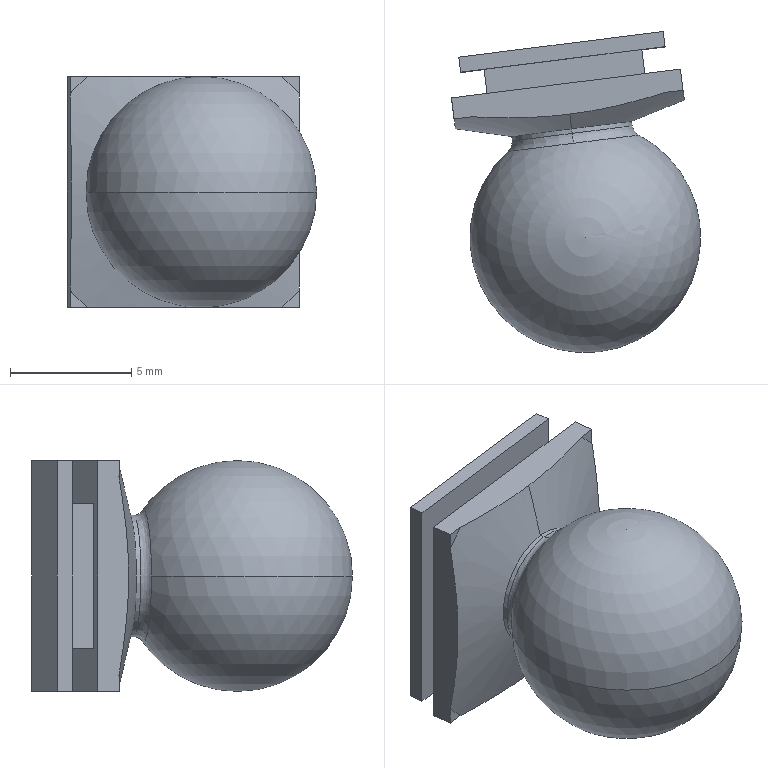Component | SolidWorks | BallJointRod-1 | 1 solid | 27 faces | box 10.26 x 13.22 x 9.5 mm | volume 678 mm3 | plane 19 | cone 2 | torus 2 | sphere 2 | cylinder 2 | commonest cylinder face diameters 5 x2
STEP:
#1=CARTESIAN_POINT('',(20.793,-12.64,5.146));
#2=VERTEX_POINT('',#1);
#3=CARTESIAN_POINT('',(20.793,-12.64,5.343));
#4=VERTEX_POINT('',#3);
#5=CARTESIAN_POINT('',(20.793,-12.64,5.245));
#6=DIRECTION('',(0.1249,-0.9922,0.));
#7=DIRECTION('',(0.,0.,-1.));
#8=AXIS2_PLACEMENT_3D('',#5,#6,#7);
#9=CIRCLE('',#8,0.09843);
#10=EDGE_CURVE('',#2,#4,#9,.T.);
#11=ORIENTED_EDGE('',*,*,#10,.F.);
#12=CARTESIAN_POINT('',(20.79,-12.616,5.058));
#13=VERTEX_POINT('',#12);
#14=CARTESIAN_POINT('',(20.788,-12.601,4.999));
#15=DIRECTION('',(-0.03232,0.2568,-0.9659));
#16=VECTOR('',#15,39.37);
#17=LINE('',#14,#16);
#18=EDGE_CURVE('',#2,#13,#17,.T.);
#19=ORIENTED_EDGE('',*,*,#18,.T.);
#20=CARTESIAN_POINT('',(20.945,-12.581,5.058));
#21=VERTEX_POINT('',#20);
#22=CARTESIAN_POINT('',(20.945,-12.581,5.058));
#23=CARTESIAN_POINT('',(20.92,-12.589,5.058));
#24=CARTESIAN_POINT('',(20.894,-12.596,5.058));
#25=CARTESIAN_POINT('',(20.842,-12.608,5.058));
#26=CARTESIAN_POINT('',(20.816,-12.613,5.058));
#27=CARTESIAN_POINT('',(20.79,-12.616,5.058));
#28=B_SPLINE_CURVE_WITH_KNOTS('',3,(#22,#23,#24,#25,#26,#27),.UNSPECIFIED.,.F.,.F.,(4,2,4),(0.,0.002023,0.004047),.UNSPECIFIED.);
#29=EDGE_CURVE('',#21,#13,#28,.T.);
#30=ORIENTED_EDGE('',*,*,#29,.F.);
#31=CARTESIAN_POINT('',(20.973,-12.577,5.086));
#32=VERTEX_POINT('',#31);
#33=CARTESIAN_POINT('',(20.788,-12.601,5.245));
#34=DIRECTION('',(-0.1249,0.9922,-0.));
#35=DIRECTION('',(-0.,-0.,-1.));
#36=AXIS2_PLACEMENT_3D('',#33,#34,#35);
#37=CIRCLE('',#36,0.2454);
#38=EDGE_CURVE('',#32,#21,#37,.T.);
#39=ORIENTED_EDGE('',*,*,#38,.F.);
#40=CARTESIAN_POINT('',(20.973,-12.577,5.403));
#41=VERTEX_POINT('',#40);
#42=CARTESIAN_POINT('',(20.973,-12.577,5.403));
#43=CARTESIAN_POINT('',(20.975,-12.586,5.351));
#44=CARTESIAN_POINT('',(20.975,-12.593,5.298));
#45=CARTESIAN_POINT('',(20.975,-12.593,5.219));
#46=CARTESIAN_POINT('',(20.975,-12.591,5.192));
#47=CARTESIAN_POINT('',(20.974,-12.586,5.139));
#48=CARTESIAN_POINT('',(20.974,-12.582,5.112));
#49=CARTESIAN_POINT('',(20.973,-12.577,5.086));
#50=B_SPLINE_CURVE_WITH_KNOTS('',3,(#42,#43,#44,#45,#46,#47,#48,#49),.UNSPECIFIED.,.F.,.F.,(4,2,2,4),(0.,0.004036,0.006054,0.008072),.UNSPECIFIED.);
#51=EDGE_CURVE('',#41,#32,#50,.T.);
#52=ORIENTED_EDGE('',*,*,#51,.F.);
#53=CARTESIAN_POINT('',(20.945,-12.581,5.432));
#54=VERTEX_POINT('',#53);
#55=CARTESIAN_POINT('',(20.788,-12.601,5.245));
#56=DIRECTION('',(-0.1249,0.9922,-0.));
#57=DIRECTION('',(-0.,-0.,-1.));
#58=AXIS2_PLACEMENT_3D('',#55,#56,#57);
#59=CIRCLE('',#58,0.2454);
#60=EDGE_CURVE('',#54,#41,#59,.T.);
#61=ORIENTED_EDGE('',*,*,#60,.F.);
#62=CARTESIAN_POINT('',(20.79,-12.616,5.432));
#63=VERTEX_POINT('',#62);
#64=CARTESIAN_POINT('',(20.79,-12.616,5.432));
#65=CARTESIAN_POINT('',(20.816,-12.613,5.432));
#66=CARTESIAN_POINT('',(20.842,-12.608,5.432));
#67=CARTESIAN_POINT('',(20.894,-12.596,5.432));
#68=CARTESIAN_POINT('',(20.92,-12.589,5.432));
#69=CARTESIAN_POINT('',(20.945,-12.581,5.432));
#70=B_SPLINE_CURVE_WITH_KNOTS('',3,(#64,#65,#66,#67,#68,#69),.UNSPECIFIED.,.F.,.F.,(4,2,4),(0.004047,0.006059,0.008072),.UNSPECIFIED.);
#71=EDGE_CURVE('',#63,#54,#70,.T.);
#72=ORIENTED_EDGE('',*,*,#71,.F.);
#73=CARTESIAN_POINT('',(20.788,-12.601,5.49));
#74=DIRECTION('',(-0.03232,0.2568,0.9659));
#75=VECTOR('',#74,39.37);
#76=LINE('',#73,#75);
#77=EDGE_CURVE('',#4,#63,#76,.T.);
#78=ORIENTED_EDGE('',*,*,#77,.F.);
#79=EDGE_LOOP('',(#11,#19,#30,#39,#52,#61,#72,#78));
#80=FACE_OUTER_BOUND('',#79,.T.);
#81=CARTESIAN_POINT('',(20.788,-12.601,5.245));
#82=DIRECTION('',(-0.1249,0.9922,-0.));
#83=DIRECTION('',(0.,0.,1.));
#84=AXIS2_PLACEMENT_3D('',#81,#82,#83);
#85=CONICAL_SURFACE('',#84,0.2454,1.309);
#86=ADVANCED_FACE('',(#80),#85,.T.);
#87=CARTESIAN_POINT('',(20.796,-12.663,5.351));
#88=VERTEX_POINT('',#87);
#89=CARTESIAN_POINT('',(20.69,-12.677,5.245));
#90=VERTEX_POINT('',#89);
#91=CARTESIAN_POINT('',(20.796,-12.663,5.245));
#92=DIRECTION('',(0.1249,-0.9922,0.));
#93=DIRECTION('',(0.,0.,-1.));
#94=AXIS2_PLACEMENT_3D('',#91,#92,#93);
#95=CIRCLE('',#94,0.1069);
#96=EDGE_CURVE('',#88,#90,#95,.T.);
#97=ORIENTED_EDGE('',*,*,#96,.F.);
#98=CARTESIAN_POINT('',(20.794,-12.647,5.343));
#99=VERTEX_POINT('',#98);
#100=CARTESIAN_POINT('',(20.794,-12.647,5.363));
#101=DIRECTION('',(0.9922,0.1249,0.));
#102=DIRECTION('',(-0.1249,0.9922,0.));
#103=AXIS2_PLACEMENT_3D('',#100,#101,#102);
#104=CIRCLE('',#103,0.01969);
#105=EDGE_CURVE('',#88,#99,#104,.T.);
#106=ORIENTED_EDGE('',*,*,#105,.T.);
#107=CARTESIAN_POINT('',(20.794,-12.647,5.146));
#108=VERTEX_POINT('',#107);
#109=CARTESIAN_POINT('',(20.794,-12.647,5.245));
#110=DIRECTION('',(-0.1249,0.9922,-0.));
#111=DIRECTION('',(0.,0.,-1.));
#112=AXIS2_PLACEMENT_3D('',#109,#110,#111);
#113=CIRCLE('',#112,0.09843);
#114=EDGE_CURVE('',#108,#99,#113,.T.);
#115=ORIENTED_EDGE('',*,*,#114,.F.);
#116=CARTESIAN_POINT('',(20.796,-12.663,5.138));
#117=VERTEX_POINT('',#116);
#118=CARTESIAN_POINT('',(20.794,-12.647,5.126));
#119=DIRECTION('',(-0.9922,-0.1249,-0.));
#120=DIRECTION('',(0.1249,-0.9922,0.));
#121=AXIS2_PLACEMENT_3D('',#118,#119,#120);
#122=CIRCLE('',#121,0.01969);
#123=EDGE_CURVE('',#117,#108,#122,.T.);
#124=ORIENTED_EDGE('',*,*,#123,.F.);
#125=CARTESIAN_POINT('',(20.796,-12.663,5.245));
#126=DIRECTION('',(0.1249,-0.9922,0.));
#127=DIRECTION('',(0.,0.,-1.));
#128=AXIS2_PLACEMENT_3D('',#125,#126,#127);
#129=CIRCLE('',#128,0.1069);
#130=EDGE_CURVE('',#90,#117,#129,.T.);
#131=ORIENTED_EDGE('',*,*,#130,.F.);
#132=EDGE_LOOP('',(#97,#106,#115,#124,#131));
#133=FACE_OUTER_BOUND('',#132,.T.);
#134=CARTESIAN_POINT('',(20.794,-12.647,5.245));
#135=DIRECTION('',(0.1249,-0.9922,0.));
#136=DIRECTION('',(0.,-0.,-1.));
#137=AXIS2_PLACEMENT_3D('',#134,#135,#136);
#138=TOROIDAL_SURFACE('',#137,0.1181,0.01969);
#139=ADVANCED_FACE('',(#133),#138,.F.);
#140=CARTESIAN_POINT('',(20.838,-13.001,5.245));
#141=VERTEX_POINT('',#140);
#142=CARTESIAN_POINT('',(20.902,-12.65,5.245));
#143=VERTEX_POINT('',#142);
#144=CARTESIAN_POINT('',(20.815,-12.815,5.245));
#145=DIRECTION('',(-0.,0.,1.));
#146=DIRECTION('',(1.,0.,0.));
#147=AXIS2_PLACEMENT_3D('',#144,#145,#146);
#148=CIRCLE('',#147,0.187);
#149=EDGE_CURVE('',#141,#143,#148,.T.);
#150=ORIENTED_EDGE('',*,*,#149,.F.);
#151=CARTESIAN_POINT('',(20.815,-12.815,5.245));
#152=DIRECTION('',(0.,-0.,-1.));
#153=DIRECTION('',(-1.,0.,0.));
#154=AXIS2_PLACEMENT_3D('',#151,#152,#153);
#155=CIRCLE('',#154,0.187);
#156=EDGE_CURVE('',#141,#90,#155,.T.);
#157=ORIENTED_EDGE('',*,*,#156,.T.);
#158=ORIENTED_EDGE('',*,*,#130,.T.);
#159=CARTESIAN_POINT('',(20.796,-12.663,5.245));
#160=DIRECTION('',(0.1249,-0.9922,0.));
#161=DIRECTION('',(0.,0.,-1.));
#162=AXIS2_PLACEMENT_3D('',#159,#160,#161);
#163=CIRCLE('',#162,0.1069);
#164=EDGE_CURVE('',#117,#143,#163,.T.);
#165=ORIENTED_EDGE('',*,*,#164,.T.);
#166=EDGE_LOOP('',(#150,#157,#158,#165));
#167=FACE_OUTER_BOUND('',#166,.T.);
#168=CARTESIAN_POINT('',(20.815,-12.815,5.245));
#169=DIRECTION('',(0.,-0.,-1.));
#170=DIRECTION('',(0.9922,0.1249,0.));
#171=AXIS2_PLACEMENT_3D('',#168,#169,#170);
#172=SPHERICAL_SURFACE('',#171,0.187);
#173=ADVANCED_FACE('',(#167),#172,.T.);
#174=ORIENTED_EDGE('',*,*,#10,.T.);
#175=CARTESIAN_POINT('',(20.788,-12.601,5.343));
#176=DIRECTION('',(0.1249,-0.9922,0.));
#177=VECTOR('',#176,39.37);
#178=LINE('',#175,#177);
#179=EDGE_CURVE('',#4,#99,#178,.T.);
#180=ORIENTED_EDGE('',*,*,#179,.T.);
#181=CARTESIAN_POINT('',(20.794,-12.647,5.245));
#182=DIRECTION('',(-0.1249,0.9922,-0.));
#183=DIRECTION('',(0.,0.,-1.));
#184=AXIS2_PLACEMENT_3D('',#181,#182,#183);
#185=CIRCLE('',#184,0.09843);
#186=EDGE_CURVE('',#99,#108,#185,.T.);
#187=ORIENTED_EDGE('',*,*,#186,.T.);
#188=CARTESIAN_POINT('',(20.788,-12.601,5.146));
#189=DIRECTION('',(0.1249,-0.9922,0.));
#190=VECTOR('',#189,39.37);
#191=LINE('',#188,#190);
#192=EDGE_CURVE('',#2,#108,#191,.T.);
#193=ORIENTED_EDGE('',*,*,#192,.F.);
#194=EDGE_LOOP('',(#174,#180,#187,#193));
#195=FACE_OUTER_BOUND('',#194,.T.);
#196=CARTESIAN_POINT('',(20.788,-12.601,5.245));
#197=DIRECTION('',(0.1249,-0.9922,0.));
#198=DIRECTION('',(0.,0.,-1.));
#199=AXIS2_PLACEMENT_3D('',#196,#197,#198);
#200=CYLINDRICAL_SURFACE('',#199,0.09843);
#201=ADVANCED_FACE('',(#195),#200,.T.);
#202=CARTESIAN_POINT('',(20.944,-12.507,5.058));
#203=VERTEX_POINT('',#202);
#204=CARTESIAN_POINT('',(20.613,-12.548,5.058));
#205=VERTEX_POINT('',#204);
#206=CARTESIAN_POINT('',(20.906,-12.511,5.058));
#207=DIRECTION('',(-0.9922,-0.1249,-0.));
#208=VECTOR('',#207,39.37);
#209=LINE('',#206,#208);
#210=EDGE_CURVE('',#203,#205,#209,.T.);
#211=ORIENTED_EDGE('',*,*,#210,.T.);
#212=CARTESIAN_POINT('',(20.61,-12.524,5.058));
#213=VERTEX_POINT('',#212);
#214=CARTESIAN_POINT('',(20.613,-12.548,5.058));
#215=DIRECTION('',(-0.1249,0.9922,-0.));
#216=VECTOR('',#215,39.37);
#217=LINE('',#214,#216);
#218=EDGE_CURVE('',#205,#213,#217,.T.);
#219=ORIENTED_EDGE('',*,*,#218,.T.);
#220=CARTESIAN_POINT('',(20.941,-12.482,5.058));
#221=VERTEX_POINT('',#220);
#222=CARTESIAN_POINT('',(20.59,-12.526,5.058));
#223=DIRECTION('',(-0.9922,-0.1249,-0.));
#224=VECTOR('',#223,39.37);
#225=LINE('',#222,#224);
#226=EDGE_CURVE('',#221,#213,#225,.T.);
#227=ORIENTED_EDGE('',*,*,#226,.F.);
#228=CARTESIAN_POINT('',(20.944,-12.507,5.058));
#229=DIRECTION('',(0.1249,-0.9922,0.));
#230=VECTOR('',#229,39.37);
#231=LINE('',#228,#230);
#232=EDGE_CURVE('',#221,#203,#231,.T.);
#233=ORIENTED_EDGE('',*,*,#232,.T.);
#234=EDGE_LOOP('',(#211,#219,#227,#233));
#235=FACE_OUTER_BOUND('',#234,.T.);
#236=CARTESIAN_POINT('',(20.59,-12.526,5.058));
#237=DIRECTION('',(-0.,0.,1.));
#238=DIRECTION('',(0.9922,0.1249,0.));
#239=AXIS2_PLACEMENT_3D('',#236,#237,#238);
#240=PLANE('',#239);
#241=ADVANCED_FACE('',(#235),#240,.F.);
#242=CARTESIAN_POINT('',(20.944,-12.507,5.432));
#243=VERTEX_POINT('',#242);
#244=CARTESIAN_POINT('',(20.613,-12.548,5.432));
#245=VERTEX_POINT('',#244);
#246=CARTESIAN_POINT('',(20.651,-12.543,5.432));
#247=DIRECTION('',(-0.9922,-0.1249,-0.));
#248=VECTOR('',#247,39.37);
#249=LINE('',#246,#248);
#250=EDGE_CURVE('',#243,#245,#249,.T.);
#251=ORIENTED_EDGE('',*,*,#250,.F.);
#252=CARTESIAN_POINT('',(20.941,-12.482,5.432));
#253=VERTEX_POINT('',#252);
#254=CARTESIAN_POINT('',(20.944,-12.507,5.432));
#255=DIRECTION('',(0.1249,-0.9922,0.));
#256=VECTOR('',#255,39.37);
#257=LINE('',#254,#256);
#258=EDGE_CURVE('',#253,#243,#257,.T.);
#259=ORIENTED_EDGE('',*,*,#258,.F.);
#260=CARTESIAN_POINT('',(20.61,-12.524,5.432));
#261=VERTEX_POINT('',#260);
#262=CARTESIAN_POINT('',(20.59,-12.526,5.432));
#263=DIRECTION('',(0.9922,0.1249,0.));
#264=VECTOR('',#263,39.37);
#265=LINE('',#262,#264);
#266=EDGE_CURVE('',#261,#253,#265,.T.);
#267=ORIENTED_EDGE('',*,*,#266,.F.);
#268=CARTESIAN_POINT('',(20.613,-12.548,5.432));
#269=DIRECTION('',(-0.1249,0.9922,-0.));
#270=VECTOR('',#269,39.37);
#271=LINE('',#268,#270);
#272=EDGE_CURVE('',#245,#261,#271,.T.);
#273=ORIENTED_EDGE('',*,*,#272,.F.);
#274=EDGE_LOOP('',(#251,#259,#267,#273));
#275=FACE_OUTER_BOUND('',#274,.T.);
#276=CARTESIAN_POINT('',(20.59,-12.526,5.432));
#277=DIRECTION('',(0.,-0.,-1.));
#278=DIRECTION('',(-0.9922,-0.1249,-0.));
#279=AXIS2_PLACEMENT_3D('',#276,#277,#278);
#280=PLANE('',#279);
#281=ADVANCED_FACE('',(#275),#280,.F.);
#282=CARTESIAN_POINT('',(20.973,-12.577,5.058));
#283=VERTEX_POINT('',#282);
#284=CARTESIAN_POINT('',(20.973,-12.577,5.432));
#285=DIRECTION('',(0.,-0.,-1.));
#286=VECTOR('',#285,39.37);
#287=LINE('',#284,#286);
#288=EDGE_CURVE('',#32,#283,#287,.T.);
#289=ORIENTED_EDGE('',*,*,#288,.F.);
#290=ORIENTED_EDGE('',*,*,#38,.T.);
#291=CARTESIAN_POINT('',(20.602,-12.624,5.058));
#292=DIRECTION('',(-0.9922,-0.1249,-0.));
#293=VECTOR('',#292,39.37);
#294=LINE('',#291,#293);
#295=EDGE_CURVE('',#283,#21,#294,.T.);
#296=ORIENTED_EDGE('',*,*,#295,.F.);
#297=EDGE_LOOP('',(#289,#290,#296));
#298=FACE_OUTER_BOUND('',#297,.T.);
#299=CARTESIAN_POINT('',(20.788,-12.601,5.245));
#300=DIRECTION('',(0.1249,-0.9922,0.));
#301=DIRECTION('',(0.,-0.,-1.));
#302=AXIS2_PLACEMENT_3D('',#299,#300,#301);
#303=PLANE('',#302);
#304=ADVANCED_FACE('',(#298),#303,.T.);
#305=CARTESIAN_POINT('',(20.63,-12.62,5.058));
#306=VERTEX_POINT('',#305);
#307=CARTESIAN_POINT('',(20.602,-12.624,5.058));
#308=VERTEX_POINT('',#307);
#309=CARTESIAN_POINT('',(20.602,-12.624,5.058));
#310=DIRECTION('',(-0.9922,-0.1249,-0.));
#311=VECTOR('',#310,39.37);
#312=LINE('',#309,#311);
#313=EDGE_CURVE('',#306,#308,#312,.T.);
#314=ORIENTED_EDGE('',*,*,#313,.F.);
#315=CARTESIAN_POINT('',(20.602,-12.624,5.086));
#316=VERTEX_POINT('',#315);
#317=CARTESIAN_POINT('',(20.788,-12.601,5.245));
#318=DIRECTION('',(-0.1249,0.9922,-0.));
#319=DIRECTION('',(0.,0.,-1.));
#320=AXIS2_PLACEMENT_3D('',#317,#318,#319);
#321=CIRCLE('',#320,0.2454);
#322=EDGE_CURVE('',#306,#316,#321,.T.);
#323=ORIENTED_EDGE('',*,*,#322,.T.);
#324=CARTESIAN_POINT('',(20.602,-12.624,5.432));
#325=DIRECTION('',(-0.,0.,1.));
#326=VECTOR('',#325,39.37);
#327=LINE('',#324,#326);
#328=EDGE_CURVE('',#308,#316,#327,.T.);
#329=ORIENTED_EDGE('',*,*,#328,.F.);
#330=EDGE_LOOP('',(#314,#323,#329));
#331=FACE_OUTER_BOUND('',#330,.T.);
#332=CARTESIAN_POINT('',(20.788,-12.601,5.245));
#333=DIRECTION('',(0.1249,-0.9922,0.));
#334=DIRECTION('',(0.,-0.,-1.));
#335=AXIS2_PLACEMENT_3D('',#332,#333,#334);
#336=PLANE('',#335);
#337=ADVANCED_FACE('',(#331),#336,.T.);
#338=CARTESIAN_POINT('',(20.602,-12.624,5.403));
#339=VERTEX_POINT('',#338);
#340=CARTESIAN_POINT('',(20.602,-12.624,5.432));
#341=VERTEX_POINT('',#340);
#342=CARTESIAN_POINT('',(20.602,-12.624,5.432));
#343=DIRECTION('',(-0.,0.,1.));
#344=VECTOR('',#343,39.37);
#345=LINE('',#342,#344);
#346=EDGE_CURVE('',#339,#341,#345,.T.);
#347=ORIENTED_EDGE('',*,*,#346,.F.);
#348=CARTESIAN_POINT('',(20.63,-12.62,5.432));
#349=VERTEX_POINT('',#348);
#350=CARTESIAN_POINT('',(20.788,-12.601,5.245));
#351=DIRECTION('',(-0.1249,0.9922,-0.));
#352=DIRECTION('',(0.,0.,-1.));
#353=AXIS2_PLACEMENT_3D('',#350,#351,#352);
#354=CIRCLE('',#353,0.2454);
#355=EDGE_CURVE('',#339,#349,#354,.T.);
#356=ORIENTED_EDGE('',*,*,#355,.T.);
#357=CARTESIAN_POINT('',(20.602,-12.624,5.432));
#358=DIRECTION('',(0.9922,0.1249,0.));
#359=VECTOR('',#358,39.37);
#360=LINE('',#357,#359);
#361=EDGE_CURVE('',#341,#349,#360,.T.);
#362=ORIENTED_EDGE('',*,*,#361,.F.);
#363=EDGE_LOOP('',(#347,#356,#362));
#364=FACE_OUTER_BOUND('',#363,.T.);
#365=CARTESIAN_POINT('',(20.788,-12.601,5.245));
#366=DIRECTION('',(0.1249,-0.9922,0.));
#367=DIRECTION('',(0.,-0.,-1.));
#368=AXIS2_PLACEMENT_3D('',#365,#366,#367);
#369=PLANE('',#368);
#370=ADVANCED_FACE('',(#364),#369,.T.);
#371=ORIENTED_EDGE('',*,*,#179,.F.);
#372=CARTESIAN_POINT('',(20.793,-12.64,5.245));
#373=DIRECTION('',(0.1249,-0.9922,0.));
#374=DIRECTION('',(0.,0.,-1.));
#375=AXIS2_PLACEMENT_3D('',#372,#373,#374);
#376=CIRCLE('',#375,0.09843);
#377=EDGE_CURVE('',#4,#2,#376,.T.);
#378=ORIENTED_EDGE('',*,*,#377,.T.);
#379=ORIENTED_EDGE('',*,*,#192,.T.);
#380=ORIENTED_EDGE('',*,*,#114,.T.);
#381=EDGE_LOOP('',(#371,#378,#379,#380));
#382=FACE_OUTER_BOUND('',#381,.T.);
#383=CARTESIAN_POINT('',(20.788,-12.601,5.245));
#384=DIRECTION('',(0.1249,-0.9922,0.));
#385=DIRECTION('',(0.,0.,-1.));
#386=AXIS2_PLACEMENT_3D('',#383,#384,#385);
#387=CYLINDRICAL_SURFACE('',#386,0.09843);
#388=ADVANCED_FACE('',(#382),#387,.T.);
#389=ORIENTED_EDGE('',*,*,#156,.F.);
#390=ORIENTED_EDGE('',*,*,#149,.T.);
#391=CARTESIAN_POINT('',(20.796,-12.663,5.245));
#392=DIRECTION('',(0.1249,-0.9922,0.));
#393=DIRECTION('',(0.,0.,-1.));
#394=AXIS2_PLACEMENT_3D('',#391,#392,#393);
#395=CIRCLE('',#394,0.1069);
#396=EDGE_CURVE('',#143,#88,#395,.T.);
#397=ORIENTED_EDGE('',*,*,#396,.T.);
#398=ORIENTED_EDGE('',*,*,#96,.T.);
#399=EDGE_LOOP('',(#389,#390,#397,#398));
#400=FACE_OUTER_BOUND('',#399,.T.);
#401=CARTESIAN_POINT('',(20.815,-12.815,5.245));
#402=DIRECTION('',(0.,-0.,-1.));
#403=DIRECTION('',(0.9922,0.1249,0.));
#404=AXIS2_PLACEMENT_3D('',#401,#402,#403);
#405=SPHERICAL_SURFACE('',#404,0.187);
#406=ADVANCED_FACE('',(#400),#405,.T.);
#407=ORIENTED_EDGE('',*,*,#105,.F.);
#408=ORIENTED_EDGE('',*,*,#396,.F.);
#409=ORIENTED_EDGE('',*,*,#164,.F.);
#410=ORIENTED_EDGE('',*,*,#123,.T.);
#411=ORIENTED_EDGE('',*,*,#186,.F.);
#412=EDGE_LOOP('',(#407,#408,#409,#410,#411));
#413=FACE_OUTER_BOUND('',#412,.T.);
#414=CARTESIAN_POINT('',(20.794,-12.647,5.245));
#415=DIRECTION('',(0.1249,-0.9922,0.));
#416=DIRECTION('',(0.,-0.,-1.));
#417=AXIS2_PLACEMENT_3D('',#414,#415,#416);
#418=TOROIDAL_SURFACE('',#417,0.1181,0.01969);
#419=ADVANCED_FACE('',(#413),#418,.F.);
#420=CARTESIAN_POINT('',(20.973,-12.577,5.432));
#421=VERTEX_POINT('',#420);
#422=CARTESIAN_POINT('',(20.602,-12.624,5.432));
#423=DIRECTION('',(0.9922,0.1249,0.));
#424=VECTOR('',#423,39.37);
#425=LINE('',#422,#424);
#426=EDGE_CURVE('',#54,#421,#425,.T.);
#427=ORIENTED_EDGE('',*,*,#426,.F.);
#428=ORIENTED_EDGE('',*,*,#60,.T.);
#429=CARTESIAN_POINT('',(20.973,-12.577,5.432));
#430=DIRECTION('',(0.,-0.,-1.));
#431=VECTOR('',#430,39.37);
#432=LINE('',#429,#431);
#433=EDGE_CURVE('',#421,#41,#432,.T.);
#434=ORIENTED_EDGE('',*,*,#433,.F.);
#435=EDGE_LOOP('',(#427,#428,#434));
#436=FACE_OUTER_BOUND('',#435,.T.);
#437=CARTESIAN_POINT('',(20.788,-12.601,5.245));
#438=DIRECTION('',(0.1249,-0.9922,0.));
#439=DIRECTION('',(0.,-0.,-1.));
#440=AXIS2_PLACEMENT_3D('',#437,#438,#439);
#441=PLANE('',#440);
#442=ADVANCED_FACE('',(#436),#441,.T.);
#443=CARTESIAN_POINT('',(20.969,-12.543,5.058));
#444=VERTEX_POINT('',#443);
#445=CARTESIAN_POINT('',(20.961,-12.48,5.058));
#446=DIRECTION('',(0.1249,-0.9922,0.));
#447=VECTOR('',#446,39.37);
#448=LINE('',#445,#447);
#449=EDGE_CURVE('',#444,#283,#448,.T.);
#450=ORIENTED_EDGE('',*,*,#449,.F.);
#451=CARTESIAN_POINT('',(20.969,-12.543,5.432));
#452=VERTEX_POINT('',#451);
#453=CARTESIAN_POINT('',(20.969,-12.543,5.058));
#454=DIRECTION('',(-0.,0.,1.));
#455=VECTOR('',#454,39.37);
#456=LINE('',#453,#455);
#457=EDGE_CURVE('',#444,#452,#456,.T.);
#458=ORIENTED_EDGE('',*,*,#457,.T.);
#459=CARTESIAN_POINT('',(20.961,-12.48,5.432));
#460=DIRECTION('',(0.1249,-0.9922,0.));
#461=VECTOR('',#460,39.37);
#462=LINE('',#459,#461);
#463=EDGE_CURVE('',#452,#421,#462,.T.);
#464=ORIENTED_EDGE('',*,*,#463,.T.);
#465=ORIENTED_EDGE('',*,*,#433,.T.);
#466=ORIENTED_EDGE('',*,*,#51,.T.);
#467=ORIENTED_EDGE('',*,*,#288,.T.);
#468=EDGE_LOOP('',(#450,#458,#464,#465,#466,#467));
#469=FACE_OUTER_BOUND('',#468,.T.);
#470=CARTESIAN_POINT('',(20.961,-12.48,5.432));
#471=DIRECTION('',(-0.9922,-0.1249,-0.));
#472=DIRECTION('',(-0.,0.,1.));
#473=AXIS2_PLACEMENT_3D('',#470,#471,#472);
#474=PLANE('',#473);
#475=ADVANCED_FACE('',(#469),#474,.F.);
#476=CARTESIAN_POINT('',(20.598,-12.59,5.058));
#477=VERTEX_POINT('',#476);
#478=CARTESIAN_POINT('',(20.59,-12.526,5.058));
#479=DIRECTION('',(0.1249,-0.9922,0.));
#480=VECTOR('',#479,39.37);
#481=LINE('',#478,#480);
#482=EDGE_CURVE('',#477,#308,#481,.T.);
#483=ORIENTED_EDGE('',*,*,#482,.F.);
#484=CARTESIAN_POINT('',(20.969,-12.543,5.058));
#485=DIRECTION('',(0.9922,0.1249,0.));
#486=VECTOR('',#485,39.37);
#487=LINE('',#484,#486);
#488=EDGE_CURVE('',#477,#444,#487,.T.);
#489=ORIENTED_EDGE('',*,*,#488,.T.);
#490=ORIENTED_EDGE('',*,*,#449,.T.);
#491=ORIENTED_EDGE('',*,*,#295,.T.);
#492=ORIENTED_EDGE('',*,*,#29,.T.);
#493=CARTESIAN_POINT('',(20.79,-12.616,5.058));
#494=CARTESIAN_POINT('',(20.764,-12.619,5.058));
#495=CARTESIAN_POINT('',(20.737,-12.621,5.058));
#496=CARTESIAN_POINT('',(20.684,-12.622,5.058));
#497=CARTESIAN_POINT('',(20.657,-12.622,5.058));
#498=CARTESIAN_POINT('',(20.63,-12.62,5.058));
#499=B_SPLINE_CURVE_WITH_KNOTS('',3,(#493,#494,#495,#496,#497,#498),.UNSPECIFIED.,.F.,.F.,(4,2,4),(0.004047,0.006059,0.008072),.UNSPECIFIED.);
#500=EDGE_CURVE('',#13,#306,#499,.T.);
#501=ORIENTED_EDGE('',*,*,#500,.T.);
#502=ORIENTED_EDGE('',*,*,#313,.T.);
#503=EDGE_LOOP('',(#483,#489,#490,#491,#492,#501,#502));
#504=FACE_OUTER_BOUND('',#503,.T.);
#505=CARTESIAN_POINT('',(20.59,-12.526,5.058));
#506=DIRECTION('',(-0.,0.,1.));
#507=DIRECTION('',(0.9922,0.1249,0.));
#508=AXIS2_PLACEMENT_3D('',#505,#506,#507);
#509=PLANE('',#508);
#510=ADVANCED_FACE('',(#504),#509,.F.);
#511=CARTESIAN_POINT('',(20.598,-12.59,5.432));
#512=VERTEX_POINT('',#511);
#513=CARTESIAN_POINT('',(20.59,-12.526,5.432));
#514=DIRECTION('',(0.1249,-0.9922,0.));
#515=VECTOR('',#514,39.37);
#516=LINE('',#513,#515);
#517=EDGE_CURVE('',#512,#341,#516,.T.);
#518=ORIENTED_EDGE('',*,*,#517,.F.);
#519=CARTESIAN_POINT('',(20.598,-12.59,5.058));
#520=DIRECTION('',(-0.,0.,1.));
#521=VECTOR('',#520,39.37);
#522=LINE('',#519,#521);
#523=EDGE_CURVE('',#477,#512,#522,.T.);
#524=ORIENTED_EDGE('',*,*,#523,.F.);
#525=ORIENTED_EDGE('',*,*,#482,.T.);
#526=ORIENTED_EDGE('',*,*,#328,.T.);
#527=CARTESIAN_POINT('',(20.602,-12.624,5.086));
#528=CARTESIAN_POINT('',(20.603,-12.633,5.138));
#529=CARTESIAN_POINT('',(20.604,-12.639,5.191));
#530=CARTESIAN_POINT('',(20.604,-12.639,5.271));
#531=CARTESIAN_POINT('',(20.604,-12.638,5.297));
#532=CARTESIAN_POINT('',(20.603,-12.632,5.35));
#533=CARTESIAN_POINT('',(20.603,-12.628,5.377));
#534=CARTESIAN_POINT('',(20.602,-12.624,5.403));
#535=B_SPLINE_CURVE_WITH_KNOTS('',3,(#527,#528,#529,#530,#531,#532,#533,#534),.UNSPECIFIED.,.F.,.F.,(4,2,2,4),(0.,0.004036,0.006054,0.008072),.UNSPECIFIED.);
#536=EDGE_CURVE('',#316,#339,#535,.T.);
#537=ORIENTED_EDGE('',*,*,#536,.T.);
#538=ORIENTED_EDGE('',*,*,#346,.T.);
#539=EDGE_LOOP('',(#518,#524,#525,#526,#537,#538));
#540=FACE_OUTER_BOUND('',#539,.T.);
#541=CARTESIAN_POINT('',(20.59,-12.526,5.432));
#542=DIRECTION('',(0.9922,0.1249,0.));
#543=DIRECTION('',(0.,-0.,-1.));
#544=AXIS2_PLACEMENT_3D('',#541,#542,#543);
#545=PLANE('',#544);
#546=ADVANCED_FACE('',(#540),#545,.F.);
#547=ORIENTED_EDGE('',*,*,#463,.F.);
#548=CARTESIAN_POINT('',(20.598,-12.59,5.432));
#549=DIRECTION('',(0.9922,0.1249,0.));
#550=VECTOR('',#549,39.37);
#551=LINE('',#548,#550);
#552=EDGE_CURVE('',#512,#452,#551,.T.);
#553=ORIENTED_EDGE('',*,*,#552,.F.);
#554=ORIENTED_EDGE('',*,*,#517,.T.);
#555=ORIENTED_EDGE('',*,*,#361,.T.);
#556=CARTESIAN_POINT('',(20.63,-12.62,5.432));
#557=CARTESIAN_POINT('',(20.657,-12.622,5.432));
#558=CARTESIAN_POINT('',(20.684,-12.622,5.432));
#559=CARTESIAN_POINT('',(20.737,-12.621,5.432));
#560=CARTESIAN_POINT('',(20.763,-12.619,5.432));
#561=CARTESIAN_POINT('',(20.79,-12.616,5.432));
#562=B_SPLINE_CURVE_WITH_KNOTS('',3,(#556,#557,#558,#559,#560,#561),.UNSPECIFIED.,.F.,.F.,(4,2,4),(0.,0.002023,0.004047),.UNSPECIFIED.);
#563=EDGE_CURVE('',#349,#63,#562,.T.);
#564=ORIENTED_EDGE('',*,*,#563,.T.);
#565=ORIENTED_EDGE('',*,*,#71,.T.);
#566=ORIENTED_EDGE('',*,*,#426,.T.);
#567=EDGE_LOOP('',(#547,#553,#554,#555,#564,#565,#566));
#568=FACE_OUTER_BOUND('',#567,.T.);
#569=CARTESIAN_POINT('',(20.59,-12.526,5.432));
#570=DIRECTION('',(0.,-0.,-1.));
#571=DIRECTION('',(-0.9922,-0.1249,-0.));
#572=AXIS2_PLACEMENT_3D('',#569,#570,#571);
#573=PLANE('',#572);
#574=ADVANCED_FACE('',(#568),#573,.F.);
#575=ORIENTED_EDGE('',*,*,#266,.T.);
#576=CARTESIAN_POINT('',(20.941,-12.482,5.058));
#577=DIRECTION('',(-0.,0.,1.));
#578=VECTOR('',#577,39.37);
#579=LINE('',#576,#578);
#580=EDGE_CURVE('',#221,#253,#579,.T.);
#581=ORIENTED_EDGE('',*,*,#580,.F.);
#582=ORIENTED_EDGE('',*,*,#226,.T.);
#583=CARTESIAN_POINT('',(20.61,-12.524,5.058));
#584=DIRECTION('',(-0.,0.,1.));
#585=VECTOR('',#584,39.37);
#586=LINE('',#583,#585);
#587=EDGE_CURVE('',#213,#261,#586,.T.);
#588=ORIENTED_EDGE('',*,*,#587,.T.);
#589=EDGE_LOOP('',(#575,#581,#582,#588));
#590=FACE_OUTER_BOUND('',#589,.T.);
#591=CARTESIAN_POINT('',(20.776,-12.503,5.245));
#592=DIRECTION('',(0.1249,-0.9922,0.));
#593=DIRECTION('',(0.,-0.,-1.));
#594=AXIS2_PLACEMENT_3D('',#591,#592,#593);
#595=PLANE('',#594);
#596=ADVANCED_FACE('',(#590),#595,.F.);
#597=ORIENTED_EDGE('',*,*,#272,.T.);
#598=ORIENTED_EDGE('',*,*,#587,.F.);
#599=ORIENTED_EDGE('',*,*,#218,.F.);
#600=CARTESIAN_POINT('',(20.613,-12.548,5.058));
#601=DIRECTION('',(-0.,0.,1.));
#602=VECTOR('',#601,39.37);
#603=LINE('',#600,#602);
#604=EDGE_CURVE('',#205,#245,#603,.T.);
#605=ORIENTED_EDGE('',*,*,#604,.T.);
#606=EDGE_LOOP('',(#597,#598,#599,#605));
#607=FACE_OUTER_BOUND('',#606,.T.);
#608=CARTESIAN_POINT('',(20.613,-12.548,5.058));
#609=DIRECTION('',(0.9922,0.1249,0.));
#610=DIRECTION('',(0.,-0.,-1.));
#611=AXIS2_PLACEMENT_3D('',#608,#609,#610);
#612=PLANE('',#611);
#613=ADVANCED_FACE('',(#607),#612,.F.);
#614=CARTESIAN_POINT('',(20.651,-12.543,5.126));
#615=VERTEX_POINT('',#614);
#616=CARTESIAN_POINT('',(20.651,-12.543,5.363));
#617=VERTEX_POINT('',#616);
#618=CARTESIAN_POINT('',(20.651,-12.543,5.058));
#619=DIRECTION('',(-0.,0.,1.));
#620=VECTOR('',#619,39.37);
#621=LINE('',#618,#620);
#622=EDGE_CURVE('',#615,#617,#621,.T.);
#623=ORIENTED_EDGE('',*,*,#622,.F.);
#624=CARTESIAN_POINT('',(20.656,-12.583,5.126));
#625=VERTEX_POINT('',#624);
#626=CARTESIAN_POINT('',(20.656,-12.583,5.126));
#627=DIRECTION('',(0.1249,-0.9922,0.));
#628=VECTOR('',#627,39.37);
#629=LINE('',#626,#628);
#630=EDGE_CURVE('',#615,#625,#629,.T.);
#631=ORIENTED_EDGE('',*,*,#630,.T.);
#632=CARTESIAN_POINT('',(20.656,-12.583,5.363));
#633=VERTEX_POINT('',#632);
#634=CARTESIAN_POINT('',(20.656,-12.583,5.058));
#635=DIRECTION('',(-0.,0.,1.));
#636=VECTOR('',#635,39.37);
#637=LINE('',#634,#636);
#638=EDGE_CURVE('',#625,#633,#637,.T.);
#639=ORIENTED_EDGE('',*,*,#638,.T.);
#640=CARTESIAN_POINT('',(20.656,-12.583,5.363));
#641=DIRECTION('',(-0.1249,0.9922,-0.));
#642=VECTOR('',#641,39.37);
#643=LINE('',#640,#642);
#644=EDGE_CURVE('',#633,#617,#643,.T.);
#645=ORIENTED_EDGE('',*,*,#644,.T.);
#646=EDGE_LOOP('',(#623,#631,#639,#645));
#647=FACE_OUTER_BOUND('',#646,.T.);
#648=CARTESIAN_POINT('',(20.656,-12.583,5.058));
#649=DIRECTION('',(0.9922,0.1249,0.));
#650=DIRECTION('',(-0.1249,0.9922,-0.));
#651=AXIS2_PLACEMENT_3D('',#648,#649,#650);
#652=PLANE('',#651);
#653=ADVANCED_FACE('',(#647),#652,.F.);
#654=ORIENTED_EDGE('',*,*,#638,.F.);
#655=CARTESIAN_POINT('',(20.911,-12.55,5.126));
#656=VERTEX_POINT('',#655);
#657=CARTESIAN_POINT('',(20.598,-12.59,5.126));
#658=DIRECTION('',(0.9922,0.1249,0.));
#659=VECTOR('',#658,39.37);
#660=LINE('',#657,#659);
#661=EDGE_CURVE('',#625,#656,#660,.T.);
#662=ORIENTED_EDGE('',*,*,#661,.T.);
#663=CARTESIAN_POINT('',(20.911,-12.55,5.363));
#664=VERTEX_POINT('',#663);
#665=CARTESIAN_POINT('',(20.911,-12.55,5.058));
#666=DIRECTION('',(-0.,0.,1.));
#667=VECTOR('',#666,39.37);
#668=LINE('',#665,#667);
#669=EDGE_CURVE('',#656,#664,#668,.T.);
#670=ORIENTED_EDGE('',*,*,#669,.T.);
#671=CARTESIAN_POINT('',(20.598,-12.59,5.363));
#672=DIRECTION('',(0.9922,0.1249,0.));
#673=VECTOR('',#672,39.37);
#674=LINE('',#671,#673);
#675=EDGE_CURVE('',#633,#664,#674,.T.);
#676=ORIENTED_EDGE('',*,*,#675,.F.);
#677=EDGE_LOOP('',(#654,#662,#670,#676));
#678=FACE_BOUND('',#677,.T.);
#679=ORIENTED_EDGE('',*,*,#488,.F.);
#680=ORIENTED_EDGE('',*,*,#523,.T.);
#681=ORIENTED_EDGE('',*,*,#552,.T.);
#682=ORIENTED_EDGE('',*,*,#457,.F.);
#683=EDGE_LOOP('',(#679,#680,#681,#682));
#684=FACE_OUTER_BOUND('',#683,.T.);
#685=CARTESIAN_POINT('',(20.969,-12.543,5.058));
#686=DIRECTION('',(0.1249,-0.9922,0.));
#687=DIRECTION('',(0.9922,0.1249,0.));
#688=AXIS2_PLACEMENT_3D('',#685,#686,#687);
#689=PLANE('',#688);
#690=ADVANCED_FACE('',(#678,#684),#689,.F.);
#691=ORIENTED_EDGE('',*,*,#669,.F.);
#692=CARTESIAN_POINT('',(20.906,-12.511,5.126));
#693=VERTEX_POINT('',#692);
#694=CARTESIAN_POINT('',(20.906,-12.511,5.126));
#695=DIRECTION('',(0.1249,-0.9922,0.));
#696=VECTOR('',#695,39.37);
#697=LINE('',#694,#696);
#698=EDGE_CURVE('',#693,#656,#697,.T.);
#699=ORIENTED_EDGE('',*,*,#698,.F.);
#700=CARTESIAN_POINT('',(20.906,-12.511,5.363));
#701=VERTEX_POINT('',#700);
#702=CARTESIAN_POINT('',(20.906,-12.511,5.058));
#703=DIRECTION('',(-0.,0.,1.));
#704=VECTOR('',#703,39.37);
#705=LINE('',#702,#704);
#706=EDGE_CURVE('',#693,#701,#705,.T.);
#707=ORIENTED_EDGE('',*,*,#706,.T.);
#708=CARTESIAN_POINT('',(20.906,-12.511,5.363));
#709=DIRECTION('',(-0.1249,0.9922,-0.));
#710=VECTOR('',#709,39.37);
#711=LINE('',#708,#710);
#712=EDGE_CURVE('',#664,#701,#711,.T.);
#713=ORIENTED_EDGE('',*,*,#712,.F.);
#714=EDGE_LOOP('',(#691,#699,#707,#713));
#715=FACE_OUTER_BOUND('',#714,.T.);
#716=CARTESIAN_POINT('',(20.911,-12.55,5.058));
#717=DIRECTION('',(-0.9922,-0.1249,-0.));
#718=DIRECTION('',(0.1249,-0.9922,0.));
#719=AXIS2_PLACEMENT_3D('',#716,#717,#718);
#720=PLANE('',#719);
#721=ADVANCED_FACE('',(#715),#720,.F.);
#722=CARTESIAN_POINT('',(20.593,-12.551,5.126));
#723=DIRECTION('',(0.9922,0.1249,0.));
#724=VECTOR('',#723,39.37);
#725=LINE('',#722,#724);
#726=EDGE_CURVE('',#615,#693,#725,.T.);
#727=ORIENTED_EDGE('',*,*,#726,.F.);
#728=ORIENTED_EDGE('',*,*,#622,.T.);
#729=CARTESIAN_POINT('',(20.593,-12.551,5.363));
#730=DIRECTION('',(0.9922,0.1249,0.));
#731=VECTOR('',#730,39.37);
#732=LINE('',#729,#731);
#733=EDGE_CURVE('',#617,#701,#732,.T.);
#734=ORIENTED_EDGE('',*,*,#733,.T.);
#735=ORIENTED_EDGE('',*,*,#706,.F.);
#736=EDGE_LOOP('',(#727,#728,#734,#735));
#737=FACE_BOUND('',#736,.T.);
#738=ORIENTED_EDGE('',*,*,#250,.T.);
#739=ORIENTED_EDGE('',*,*,#604,.F.);
#740=ORIENTED_EDGE('',*,*,#210,.F.);
#741=CARTESIAN_POINT('',(20.944,-12.507,5.058));
#742=DIRECTION('',(-0.,0.,1.));
#743=VECTOR('',#742,39.37);
#744=LINE('',#741,#743);
#745=EDGE_CURVE('',#203,#243,#744,.T.);
#746=ORIENTED_EDGE('',*,*,#745,.T.);
#747=EDGE_LOOP('',(#738,#739,#740,#746));
#748=FACE_OUTER_BOUND('',#747,.T.);
#749=CARTESIAN_POINT('',(20.906,-12.511,5.058));
#750=DIRECTION('',(-0.1249,0.9922,-0.));
#751=DIRECTION('',(-0.9922,-0.1249,-0.));
#752=AXIS2_PLACEMENT_3D('',#749,#750,#751);
#753=PLANE('',#752);
#754=ADVANCED_FACE('',(#737,#748),#753,.F.);
#755=ORIENTED_EDGE('',*,*,#258,.T.);
#756=ORIENTED_EDGE('',*,*,#745,.F.);
#757=ORIENTED_EDGE('',*,*,#232,.F.);
#758=ORIENTED_EDGE('',*,*,#580,.T.);
#759=EDGE_LOOP('',(#755,#756,#757,#758));
#760=FACE_OUTER_BOUND('',#759,.T.);
#761=CARTESIAN_POINT('',(20.944,-12.507,5.058));
#762=DIRECTION('',(-0.9922,-0.1249,-0.));
#763=DIRECTION('',(-0.,0.,1.));
#764=AXIS2_PLACEMENT_3D('',#761,#762,#763);
#765=PLANE('',#764);
#766=ADVANCED_FACE('',(#760),#765,.F.);
#767=ORIENTED_EDGE('',*,*,#18,.F.);
#768=ORIENTED_EDGE('',*,*,#377,.F.);
#769=ORIENTED_EDGE('',*,*,#77,.T.);
#770=ORIENTED_EDGE('',*,*,#563,.F.);
#771=ORIENTED_EDGE('',*,*,#355,.F.);
#772=ORIENTED_EDGE('',*,*,#536,.F.);
#773=ORIENTED_EDGE('',*,*,#322,.F.);
#774=ORIENTED_EDGE('',*,*,#500,.F.);
#775=EDGE_LOOP('',(#767,#768,#769,#770,#771,#772,#773,#774));
#776=FACE_OUTER_BOUND('',#775,.T.);
#777=CARTESIAN_POINT('',(20.788,-12.601,5.245));
#778=DIRECTION('',(-0.1249,0.9922,-0.));
#779=DIRECTION('',(0.,0.,1.));
#780=AXIS2_PLACEMENT_3D('',#777,#778,#779);
#781=CONICAL_SURFACE('',#780,0.2454,1.309);
#782=ADVANCED_FACE('',(#776),#781,.T.);
#783=ORIENTED_EDGE('',*,*,#675,.T.);
#784=ORIENTED_EDGE('',*,*,#712,.T.);
#785=ORIENTED_EDGE('',*,*,#733,.F.);
#786=ORIENTED_EDGE('',*,*,#644,.F.);
#787=EDGE_LOOP('',(#783,#784,#785,#786));
#788=FACE_OUTER_BOUND('',#787,.T.);
#789=CARTESIAN_POINT('',(20.593,-12.551,5.363));
#790=DIRECTION('',(0.,-0.,-1.));
#791=DIRECTION('',(-0.9922,-0.1249,-0.));
#792=AXIS2_PLACEMENT_3D('',#789,#790,#791);
#793=PLANE('',#792);
#794=ADVANCED_FACE('',(#788),#793,.F.);
#795=ORIENTED_EDGE('',*,*,#726,.T.);
#796=ORIENTED_EDGE('',*,*,#698,.T.);
#797=ORIENTED_EDGE('',*,*,#661,.F.);
#798=ORIENTED_EDGE('',*,*,#630,.F.);
#799=EDGE_LOOP('',(#795,#796,#797,#798));
#800=FACE_OUTER_BOUND('',#799,.T.);
#801=CARTESIAN_POINT('',(20.593,-12.551,5.126));
#802=DIRECTION('',(-0.,0.,1.));
#803=DIRECTION('',(0.9922,0.1249,0.));
#804=AXIS2_PLACEMENT_3D('',#801,#802,#803);
#805=PLANE('',#804);
#806=ADVANCED_FACE('',(#800),#805,.F.);
#807=CLOSED_SHELL('',(#86,#139,#173,#201,#241,#281,#304,#337,#370,#388,#406,#419,#442,#475,#510,#546,#574,#596,#613,#653,#690,#721,#754,#766,#782,#794,#806));
#808=MANIFOLD_SOLID_BREP('',#807);
#809=CARTESIAN_POINT('',(0.,0.,0.));
#810=DIRECTION('',(0.,0.,1.));
#811=DIRECTION('',(1.,0.,0.));
#812=AXIS2_PLACEMENT_3D('',#809,#810,#811);
#813=(LENGTH_UNIT()NAMED_UNIT(*)SI_UNIT($,.METRE.));
#814=LENGTH_MEASURE_WITH_UNIT(LENGTH_MEASURE(0.0254),#813);
#815=DIMENSIONAL_EXPONENTS(1.,0.,0.,0.,0.,0.,0.);
#816=(CONVERSION_BASED_UNIT('',#814)LENGTH_UNIT()NAMED_UNIT(#815));
#817=UNCERTAINTY_MEASURE_WITH_UNIT(LENGTH_MEASURE(0.00001),#816,'','');
#818=(NAMED_UNIT(*)PLANE_ANGLE_UNIT()SI_UNIT($,.RADIAN.));
#819=(NAMED_UNIT(*)SI_UNIT($,.STERADIAN.)SOLID_ANGLE_UNIT());
#820=(GEOMETRIC_REPRESENTATION_CONTEXT(3)GLOBAL_UNCERTAINTY_ASSIGNED_CONTEXT((#817))GLOBAL_UNIT_ASSIGNED_CONTEXT((#816,#818,#819))REPRESENTATION_CONTEXT('',''));
#821=ADVANCED_BREP_SHAPE_REPRESENTATION('',(#808,#812),#820);
#822=COLOUR_RGB('',0.7922,0.8196,0.9333);
#823=FILL_AREA_STYLE_COLOUR('',#822);
#824=FILL_AREA_STYLE('',(#823));
#825=SURFACE_STYLE_FILL_AREA(#824);
#826=SURFACE_SIDE_STYLE('',(#825));
#827=SURFACE_STYLE_USAGE(.BOTH.,#826);
#828=PRESENTATION_STYLE_ASSIGNMENT((#827));
#829=STYLED_ITEM('',(#828),#808);
#830=(LENGTH_UNIT()NAMED_UNIT(*)SI_UNIT($,.METRE.));
#831=LENGTH_MEASURE_WITH_UNIT(LENGTH_MEASURE(0.0254),#830);
#832=DIMENSIONAL_EXPONENTS(1.,0.,0.,0.,0.,0.,0.);
#833=(CONVERSION_BASED_UNIT('',#831)LENGTH_UNIT()NAMED_UNIT(#832));
#834=UNCERTAINTY_MEASURE_WITH_UNIT(LENGTH_MEASURE(0.00001),#833,'','');
#835=(NAMED_UNIT(*)PLANE_ANGLE_UNIT()SI_UNIT($,.RADIAN.));
#836=(NAMED_UNIT(*)SI_UNIT($,.STERADIAN.)SOLID_ANGLE_UNIT());
#837=(GEOMETRIC_REPRESENTATION_CONTEXT(3)GLOBAL_UNCERTAINTY_ASSIGNED_CONTEXT((#834))GLOBAL_UNIT_ASSIGNED_CONTEXT((#833,#835,#836))REPRESENTATION_CONTEXT('',''));
#838=MECHANICAL_DESIGN_GEOMETRIC_PRESENTATION_REPRESENTATION('',(#829),#837);
#839=PRESENTATION_LAYER_ASSIGNMENT('','',(#829));